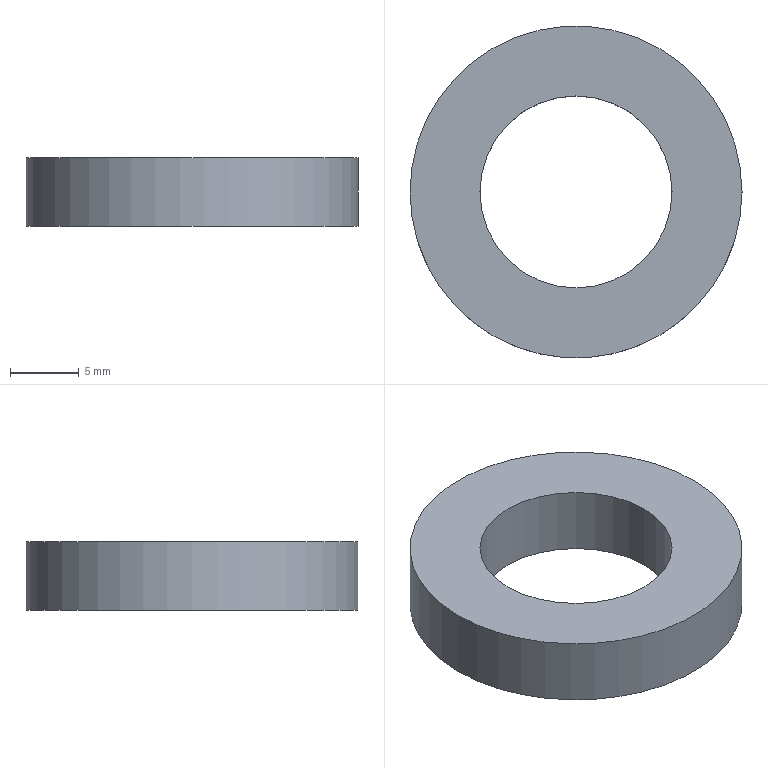Component | NX | PISTON_RING | 1 solid | 4 faces | box 24.2 x 24.2 x 5 mm | volume 1530 mm3 | cylinder 2 | plane 2 | commonest cylinder face diameters 24.2 x1 14 x1
STEP:
#1=CARTESIAN_POINT('',(0.,0.,0.));
#2=DIRECTION('',(0.,0.,1.));
#3=DIRECTION('',(1.,0.,0.));
#4=AXIS2_PLACEMENT_3D('',#1,#2,#3);
#5=CARTESIAN_POINT('',(12.1,-10.,157.621));
#6=VERTEX_POINT('',#5);
#7=CARTESIAN_POINT('',(-0.,-10.,157.621));
#8=DIRECTION('',(0.,0.,-1.));
#9=DIRECTION('',(1.,0.,0.));
#10=AXIS2_PLACEMENT_3D('',#7,#8,#9);
#11=CIRCLE('',#10,12.1);
#12=CARTESIAN_POINT('',(-0.,-10.,157.621));
#13=DIRECTION('',(0.,0.,-1.));
#14=DIRECTION('',(-1.,0.,0.));
#15=AXIS2_PLACEMENT_3D('',#12,#13,#14);
#16=CYLINDRICAL_SURFACE('',#15,12.1);
#17=CARTESIAN_POINT('',(3.142,0.));
#18=DIRECTION('',(1.,0.));
#19=VECTOR('',#18,1.);
#20=LINE('',#17,#19);
#21=(GEOMETRIC_REPRESENTATION_CONTEXT(2)PARAMETRIC_REPRESENTATION_CONTEXT()REPRESENTATION_CONTEXT('',''));
#22=DEFINITIONAL_REPRESENTATION('',(#20),#21);
#23=PCURVE('',#16,#22);
#24=CARTESIAN_POINT('',(-0.,-10.,157.621));
#25=DIRECTION('',(0.,0.,-1.));
#26=DIRECTION('',(-1.,0.,0.));
#27=AXIS2_PLACEMENT_3D('',#24,#25,#26);
#28=PLANE('',#27);
#29=CARTESIAN_POINT('',(0.,0.));
#30=DIRECTION('',(-1.,0.));
#31=AXIS2_PLACEMENT_2D('',#29,#30);
#32=CIRCLE('',#31,12.1);
#33=(GEOMETRIC_REPRESENTATION_CONTEXT(2)PARAMETRIC_REPRESENTATION_CONTEXT()REPRESENTATION_CONTEXT('',''));
#34=DEFINITIONAL_REPRESENTATION('',(#32),#33);
#35=PCURVE('',#28,#34);
#36=SURFACE_CURVE('',#11,(#23,#35),.PCURVE_S1.);
#37=EDGE_CURVE('',#6,#6,#36,.T.);
#38=ORIENTED_EDGE('',*,*,#37,.T.);
#39=CARTESIAN_POINT('',(12.1,-10.,152.621));
#40=VERTEX_POINT('',#39);
#41=CARTESIAN_POINT('',(12.1,-10.,157.621));
#42=CARTESIAN_POINT('',(12.1,-10.,152.621));
#43=B_SPLINE_CURVE_WITH_KNOTS('',1,(#41,#42),.UNSPECIFIED.,.F.,.F.,(2,2),(0.,5.),.PIECEWISE_BEZIER_KNOTS.);
#44=CARTESIAN_POINT('',(9.425,0.));
#45=DIRECTION('',(0.,1.));
#46=VECTOR('',#45,1.);
#47=LINE('',#44,#46);
#48=(GEOMETRIC_REPRESENTATION_CONTEXT(2)PARAMETRIC_REPRESENTATION_CONTEXT()REPRESENTATION_CONTEXT('',''));
#49=DEFINITIONAL_REPRESENTATION('',(#47),#48);
#50=PCURVE('',#16,#49);
#51=CARTESIAN_POINT('',(3.142,0.));
#52=DIRECTION('',(0.,1.));
#53=VECTOR('',#52,1.);
#54=LINE('',#51,#53);
#55=(GEOMETRIC_REPRESENTATION_CONTEXT(2)PARAMETRIC_REPRESENTATION_CONTEXT()REPRESENTATION_CONTEXT('',''));
#56=DEFINITIONAL_REPRESENTATION('',(#54),#55);
#57=PCURVE('',#16,#56);
#58=SEAM_CURVE('',#43,(#50,#57),.PCURVE_S1.);
#59=EDGE_CURVE('',#6,#40,#58,.T.);
#60=ORIENTED_EDGE('',*,*,#59,.T.);
#61=CARTESIAN_POINT('',(-0.,-10.,152.621));
#62=DIRECTION('',(0.,0.,-1.));
#63=DIRECTION('',(1.,0.,0.));
#64=AXIS2_PLACEMENT_3D('',#61,#62,#63);
#65=CIRCLE('',#64,12.1);
#66=CARTESIAN_POINT('',(3.142,5.));
#67=DIRECTION('',(1.,0.));
#68=VECTOR('',#67,1.);
#69=LINE('',#66,#68);
#70=(GEOMETRIC_REPRESENTATION_CONTEXT(2)PARAMETRIC_REPRESENTATION_CONTEXT()REPRESENTATION_CONTEXT('',''));
#71=DEFINITIONAL_REPRESENTATION('',(#69),#70);
#72=PCURVE('',#16,#71);
#73=CARTESIAN_POINT('',(-0.,-10.,152.621));
#74=DIRECTION('',(0.,0.,-1.));
#75=DIRECTION('',(-1.,0.,0.));
#76=AXIS2_PLACEMENT_3D('',#73,#74,#75);
#77=PLANE('',#76);
#78=CARTESIAN_POINT('',(0.,0.));
#79=DIRECTION('',(-1.,0.));
#80=AXIS2_PLACEMENT_2D('',#78,#79);
#81=CIRCLE('',#80,12.1);
#82=(GEOMETRIC_REPRESENTATION_CONTEXT(2)PARAMETRIC_REPRESENTATION_CONTEXT()REPRESENTATION_CONTEXT('',''));
#83=DEFINITIONAL_REPRESENTATION('',(#81),#82);
#84=PCURVE('',#77,#83);
#85=SURFACE_CURVE('',#65,(#72,#84),.PCURVE_S1.);
#86=EDGE_CURVE('',#40,#40,#85,.T.);
#87=ORIENTED_EDGE('',*,*,#86,.F.);
#88=ORIENTED_EDGE('',*,*,#59,.F.);
#89=EDGE_LOOP('',(#38,#60,#87,#88));
#90=FACE_BOUND('',#89,.T.);
#91=ADVANCED_FACE('',(#90),#16,.T.);
#92=CARTESIAN_POINT('',(7.,-10.,157.621));
#93=VERTEX_POINT('',#92);
#94=CARTESIAN_POINT('',(-0.,-10.,157.621));
#95=DIRECTION('',(0.,0.,-1.));
#96=DIRECTION('',(1.,0.,0.));
#97=AXIS2_PLACEMENT_3D('',#94,#95,#96);
#98=CIRCLE('',#97,7.);
#99=CARTESIAN_POINT('',(-0.,-10.,157.621));
#100=DIRECTION('',(0.,0.,-1.));
#101=DIRECTION('',(-1.,0.,0.));
#102=AXIS2_PLACEMENT_3D('',#99,#100,#101);
#103=CYLINDRICAL_SURFACE('',#102,7.);
#104=CARTESIAN_POINT('',(3.142,0.));
#105=DIRECTION('',(1.,0.));
#106=VECTOR('',#105,1.);
#107=LINE('',#104,#106);
#108=(GEOMETRIC_REPRESENTATION_CONTEXT(2)PARAMETRIC_REPRESENTATION_CONTEXT()REPRESENTATION_CONTEXT('',''));
#109=DEFINITIONAL_REPRESENTATION('',(#107),#108);
#110=PCURVE('',#103,#109);
#111=CARTESIAN_POINT('',(0.,0.));
#112=DIRECTION('',(-1.,0.));
#113=AXIS2_PLACEMENT_2D('',#111,#112);
#114=CIRCLE('',#113,7.);
#115=(GEOMETRIC_REPRESENTATION_CONTEXT(2)PARAMETRIC_REPRESENTATION_CONTEXT()REPRESENTATION_CONTEXT('',''));
#116=DEFINITIONAL_REPRESENTATION('',(#114),#115);
#117=PCURVE('',#28,#116);
#118=SURFACE_CURVE('',#98,(#110,#117),.PCURVE_S1.);
#119=EDGE_CURVE('',#93,#93,#118,.T.);
#120=ORIENTED_EDGE('',*,*,#119,.T.);
#121=CARTESIAN_POINT('',(7.,-10.,152.621));
#122=VERTEX_POINT('',#121);
#123=CARTESIAN_POINT('',(7.,-10.,157.621));
#124=CARTESIAN_POINT('',(7.,-10.,152.621));
#125=B_SPLINE_CURVE_WITH_KNOTS('',1,(#123,#124),.UNSPECIFIED.,.F.,.F.,(2,2),(0.,5.),.PIECEWISE_BEZIER_KNOTS.);
#126=CARTESIAN_POINT('',(9.425,0.));
#127=DIRECTION('',(0.,1.));
#128=VECTOR('',#127,1.);
#129=LINE('',#126,#128);
#130=(GEOMETRIC_REPRESENTATION_CONTEXT(2)PARAMETRIC_REPRESENTATION_CONTEXT()REPRESENTATION_CONTEXT('',''));
#131=DEFINITIONAL_REPRESENTATION('',(#129),#130);
#132=PCURVE('',#103,#131);
#133=CARTESIAN_POINT('',(3.142,0.));
#134=DIRECTION('',(0.,1.));
#135=VECTOR('',#134,1.);
#136=LINE('',#133,#135);
#137=(GEOMETRIC_REPRESENTATION_CONTEXT(2)PARAMETRIC_REPRESENTATION_CONTEXT()REPRESENTATION_CONTEXT('',''));
#138=DEFINITIONAL_REPRESENTATION('',(#136),#137);
#139=PCURVE('',#103,#138);
#140=SEAM_CURVE('',#125,(#132,#139),.PCURVE_S1.);
#141=EDGE_CURVE('',#93,#122,#140,.T.);
#142=ORIENTED_EDGE('',*,*,#141,.T.);
#143=CARTESIAN_POINT('',(-0.,-10.,152.621));
#144=DIRECTION('',(0.,0.,-1.));
#145=DIRECTION('',(1.,0.,0.));
#146=AXIS2_PLACEMENT_3D('',#143,#144,#145);
#147=CIRCLE('',#146,7.);
#148=CARTESIAN_POINT('',(3.142,5.));
#149=DIRECTION('',(1.,0.));
#150=VECTOR('',#149,1.);
#151=LINE('',#148,#150);
#152=(GEOMETRIC_REPRESENTATION_CONTEXT(2)PARAMETRIC_REPRESENTATION_CONTEXT()REPRESENTATION_CONTEXT('',''));
#153=DEFINITIONAL_REPRESENTATION('',(#151),#152);
#154=PCURVE('',#103,#153);
#155=CARTESIAN_POINT('',(0.,0.));
#156=DIRECTION('',(-1.,0.));
#157=AXIS2_PLACEMENT_2D('',#155,#156);
#158=CIRCLE('',#157,7.);
#159=(GEOMETRIC_REPRESENTATION_CONTEXT(2)PARAMETRIC_REPRESENTATION_CONTEXT()REPRESENTATION_CONTEXT('',''));
#160=DEFINITIONAL_REPRESENTATION('',(#158),#159);
#161=PCURVE('',#77,#160);
#162=SURFACE_CURVE('',#147,(#154,#161),.PCURVE_S1.);
#163=EDGE_CURVE('',#122,#122,#162,.T.);
#164=ORIENTED_EDGE('',*,*,#163,.F.);
#165=ORIENTED_EDGE('',*,*,#141,.F.);
#166=EDGE_LOOP('',(#120,#142,#164,#165));
#167=FACE_BOUND('',#166,.F.);
#168=ADVANCED_FACE('',(#167),#103,.F.);
#169=ORIENTED_EDGE('',*,*,#37,.F.);
#170=EDGE_LOOP('',(#169));
#171=FACE_BOUND('',#170,.T.);
#172=ORIENTED_EDGE('',*,*,#119,.T.);
#173=EDGE_LOOP('',(#172));
#174=FACE_BOUND('',#173,.T.);
#175=ADVANCED_FACE('',(#171,#174),#28,.F.);
#176=ORIENTED_EDGE('',*,*,#86,.T.);
#177=EDGE_LOOP('',(#176));
#178=FACE_BOUND('',#177,.T.);
#179=ORIENTED_EDGE('',*,*,#163,.F.);
#180=EDGE_LOOP('',(#179));
#181=FACE_BOUND('',#180,.T.);
#182=ADVANCED_FACE('',(#178,#181),#77,.T.);
#183=CLOSED_SHELL('',(#91,#168,#175,#182));
#184=MANIFOLD_SOLID_BREP('',#183);
#185=(LENGTH_UNIT()NAMED_UNIT(*)SI_UNIT(.MILLI.,.METRE.));
#186=UNCERTAINTY_MEASURE_WITH_UNIT(LENGTH_MEASURE(0.00001),#185,'','');
#187=(NAMED_UNIT(*)PLANE_ANGLE_UNIT()SI_UNIT($,.RADIAN.));
#188=(NAMED_UNIT(*)SI_UNIT($,.STERADIAN.)SOLID_ANGLE_UNIT());
#189=(GEOMETRIC_REPRESENTATION_CONTEXT(3)GLOBAL_UNCERTAINTY_ASSIGNED_CONTEXT((#186))GLOBAL_UNIT_ASSIGNED_CONTEXT((#185,#187,#188))REPRESENTATION_CONTEXT('',''));
#190=ADVANCED_BREP_SHAPE_REPRESENTATION('',(#4,#184),#189);